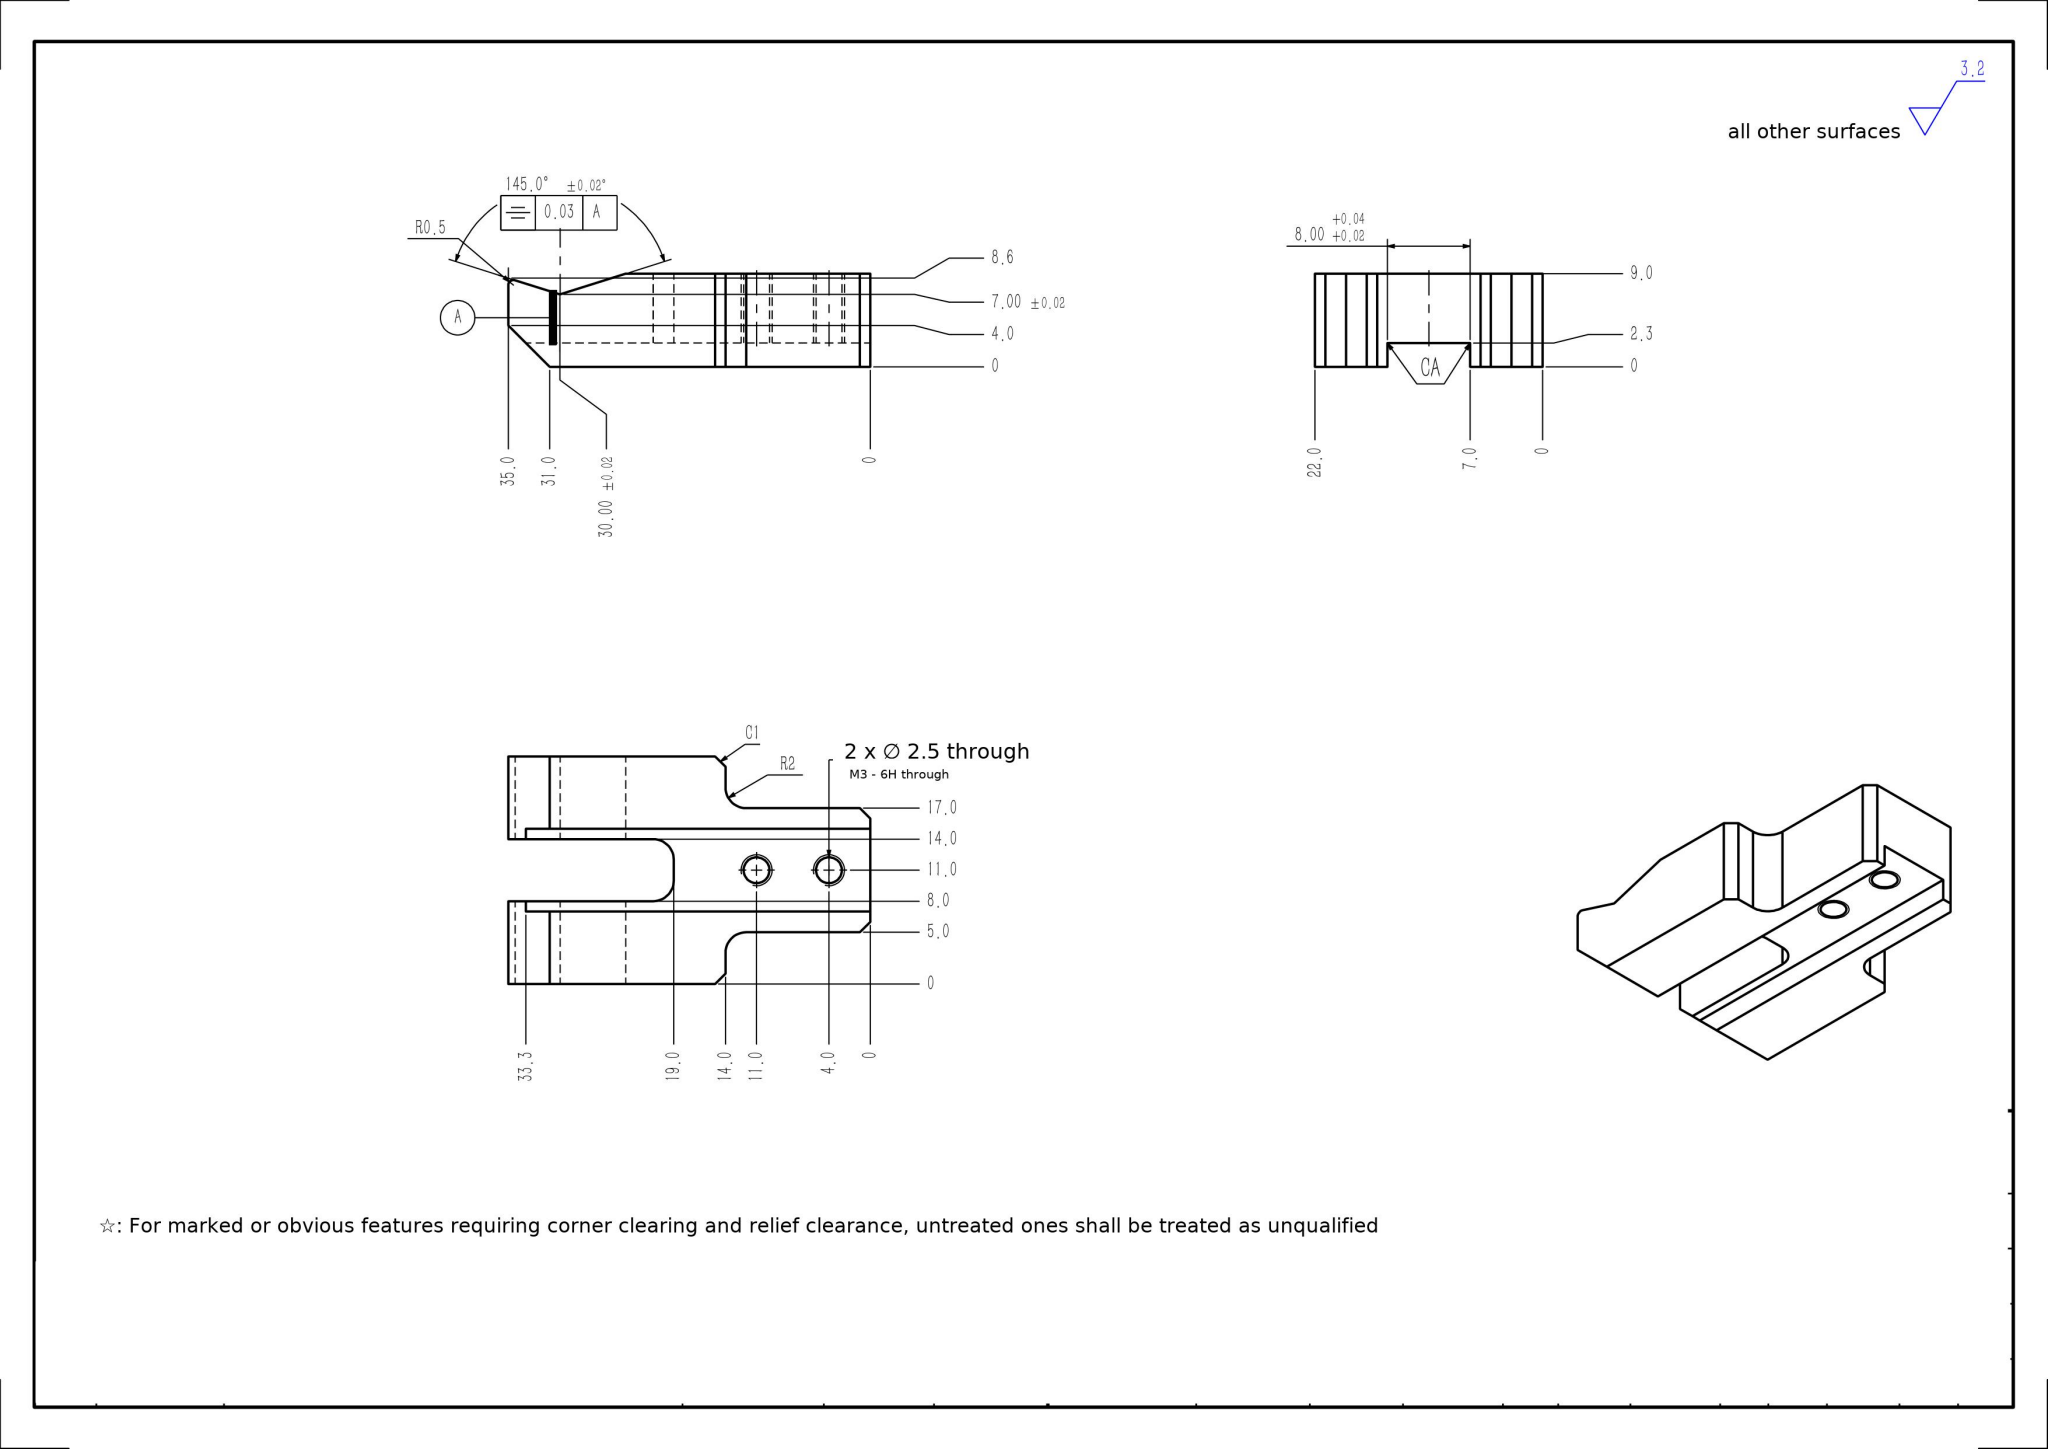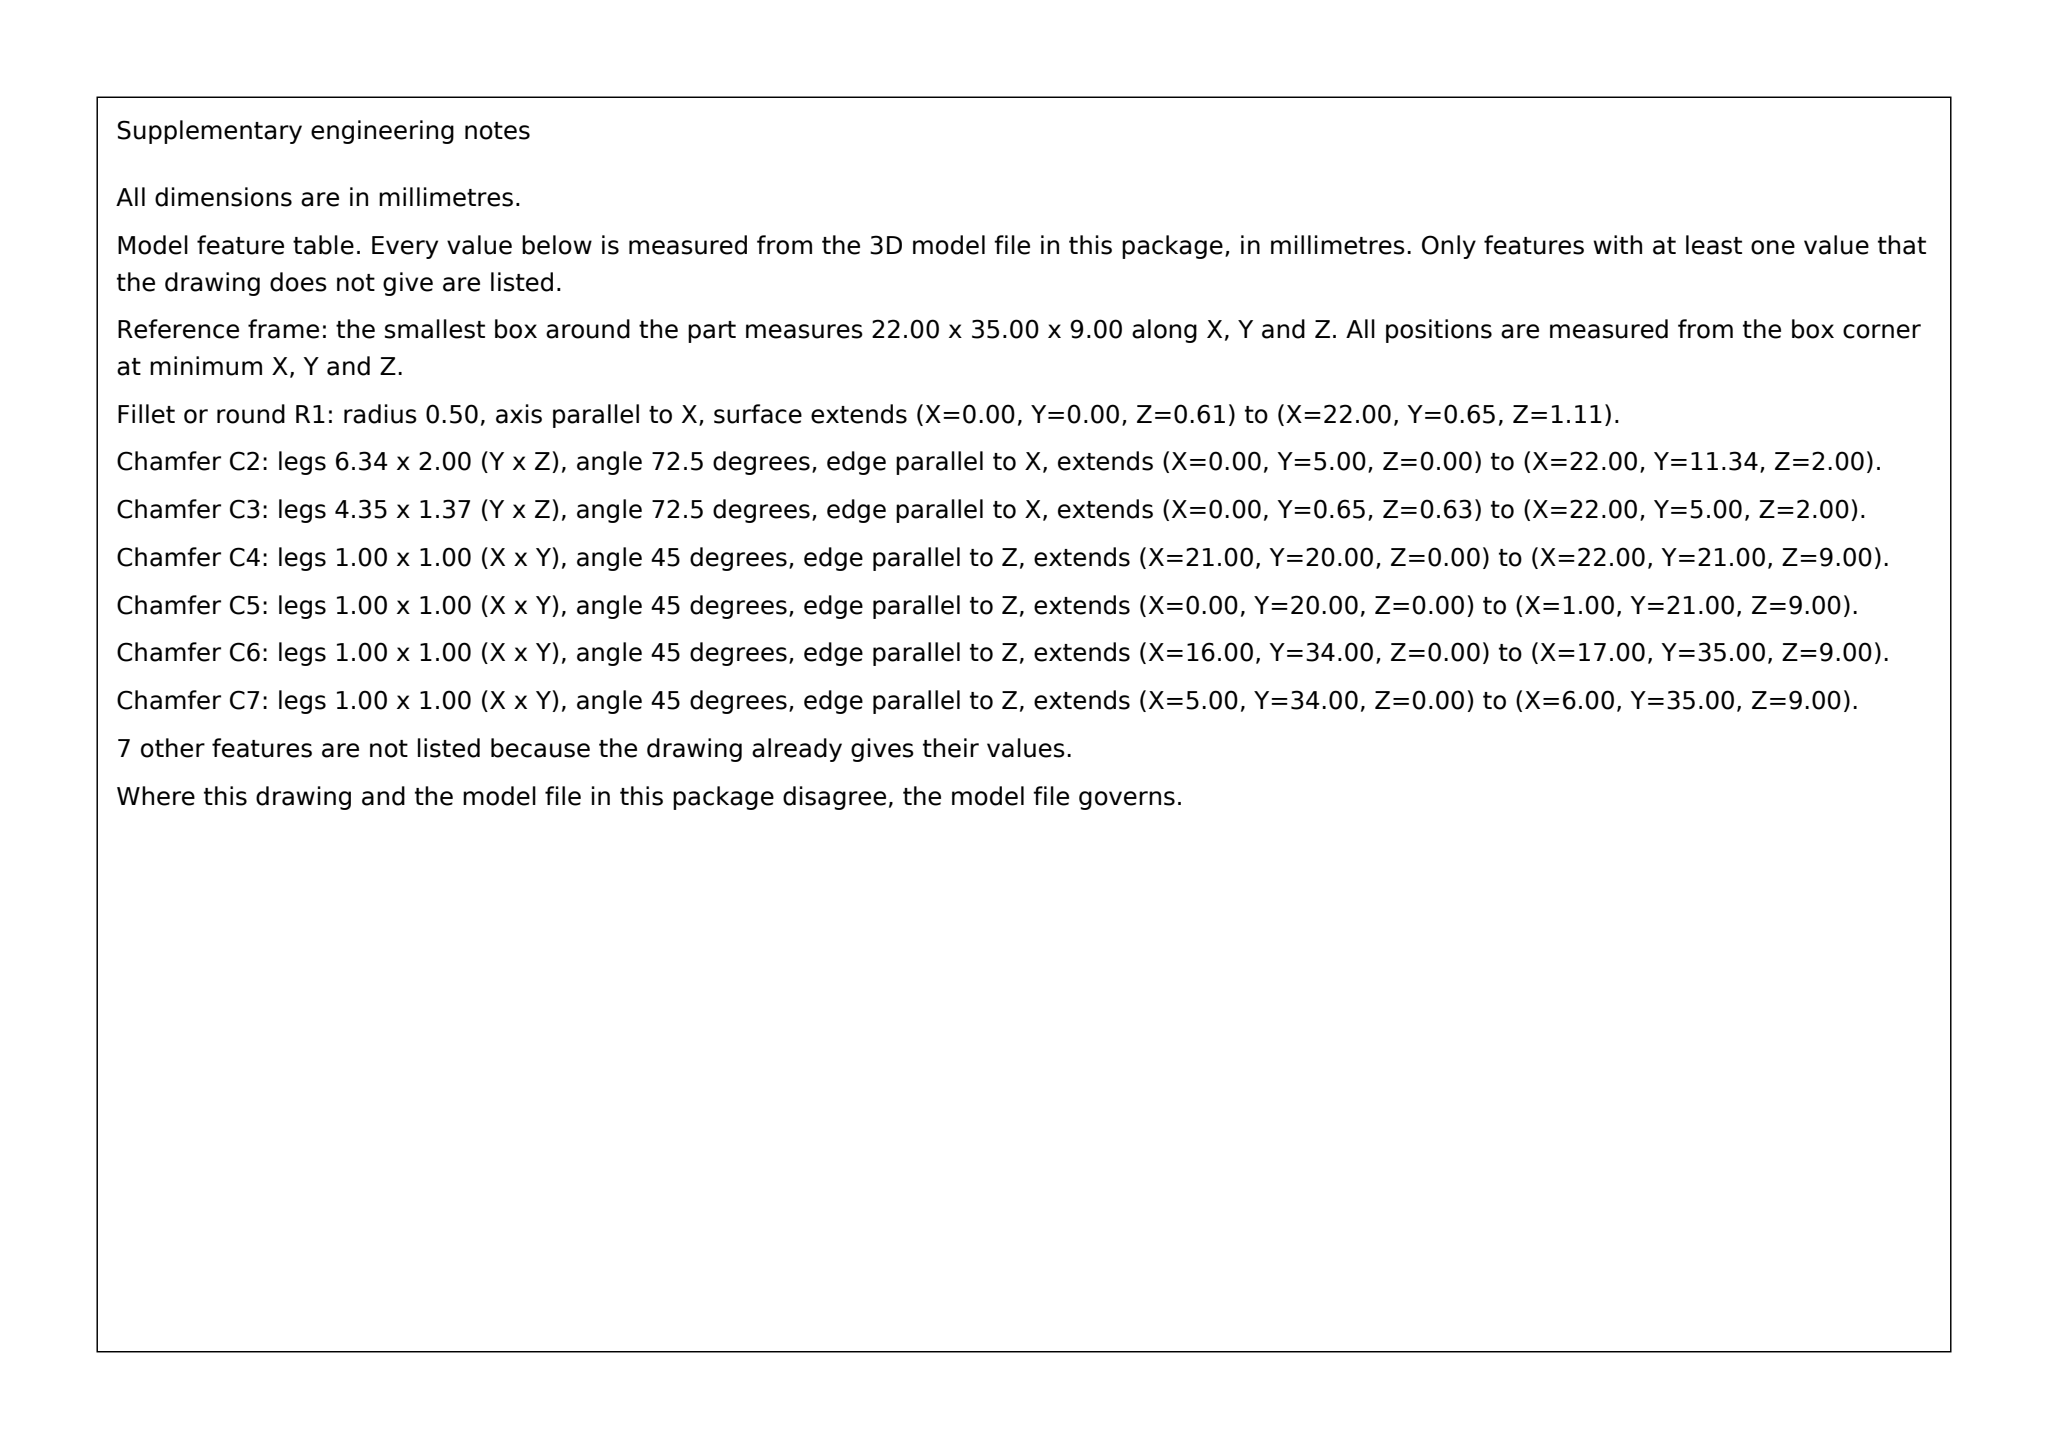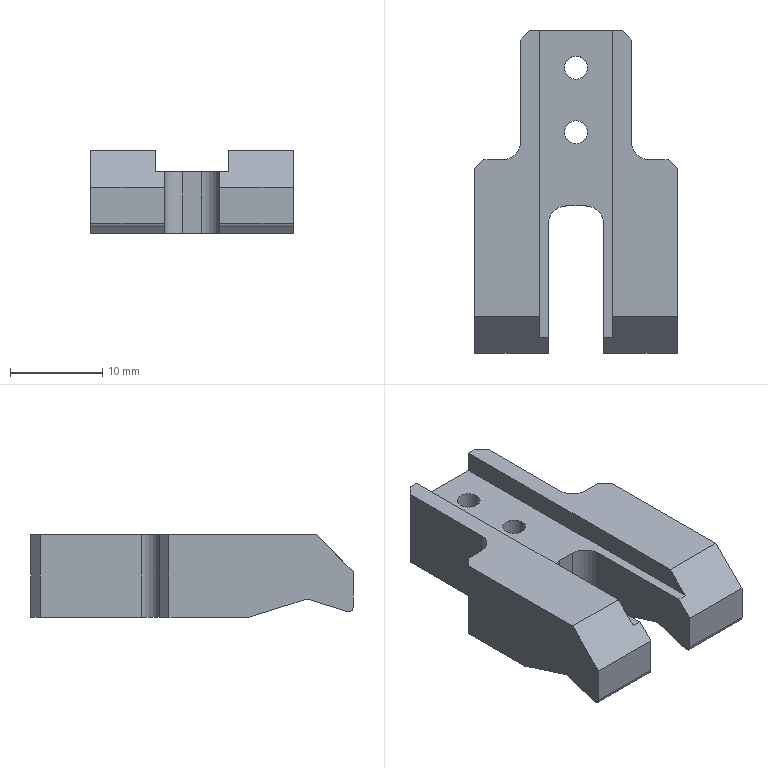Part | SolidWorks | mm | 1 solid | 40 faces | box 22 x 35 x 9 mm | volume 4011 mm3 | plane 28 | cylinder 12 | commonest cylinder face diameters 1 x4 2.5 x4 4 x4
build123d program:
from build123d import *

# Parameters (mm, degrees)
SKETCH1_W           = 22
SKETCH1_H           = 35
BOSS_EXTRUDE1_DEPTH = 9
SKETCH2_W           = 6
SKETCH2_H           = 16
CUT_EXTRUDE1_DEPTH  = 43.308
CUT_EXTRUDE2_DEPTH  = 43.308
SKETCH4_W           = 8
SKETCH4_H           = 42.52
CUT_EXTRUDE3_DEPTH  = 2.3
M3_TAPPED_HOLE1_D   = 2.5
SKETCH7_W           = 5
SKETCH7_H           = 14
CUT_EXTRUDE4_DEPTH  = 43.308
FILLET1_SIZE        = 1
CHAMFER1_SIZE       = 1
CHAMFER2_SIZE       = 4
FILLET2_R           = 2
FILLET3_R           = 2
FILLET4_R           = 0.5


with BuildPart() as part:
    # Sketch1 → Boss-Extrude1 (new body)
    with BuildSketch(Plane.XY):
        with Locations((11, -17.5)):
            Rectangle(SKETCH1_W, SKETCH1_H)
    extrude(amount=BOSS_EXTRUDE1_DEPTH)

    # Sketch2 → Cut-Extrude1 (cut, through all)
    with BuildSketch(Plane.XY.offset(9)):
        with Locations((11, -27)):
            Rectangle(SKETCH2_W, SKETCH2_H)
    extrude(amount=-CUT_EXTRUDE1_DEPTH, mode=Mode.SUBTRACT)

    # Sketch3 → Cut-Extrude2 (cut, through all)
    with BuildSketch(Plane(origin=(22, 0, 0), x_dir=(0, 0, -1), z_dir=(1, 0, 0))):
        Polygon((0, -23.657), (-2, -30), (0, -36.343), align=None)
    extrude(amount=-CUT_EXTRUDE2_DEPTH, mode=Mode.SUBTRACT)

    # Sketch4 → Cut-Extrude3 (cut)
    with BuildSketch(Plane.XY.offset(9)):
        with Locations((11, -21.26)):
            Rectangle(SKETCH4_W, SKETCH4_H)
    extrude(amount=-CUT_EXTRUDE3_DEPTH, mode=Mode.SUBTRACT)

    # M3 Tapped Hole1 (through all)
    with Locations(Plane.XY.offset(6.7)):
        with Locations((11, -4), (11, -11)):
            Hole(M3_TAPPED_HOLE1_D / 2)

    # Sketch7 → Cut-Extrude4 (cut, through all)
    with BuildSketch(Plane.XY.offset(9)):
        with Locations((19.5, -7)):
            Rectangle(SKETCH7_W, SKETCH7_H)
        with Locations((2.5, -7)):
            Rectangle(SKETCH7_W, SKETCH7_H)
    extrude(amount=-CUT_EXTRUDE4_DEPTH, mode=Mode.SUBTRACT)

    # Fillet1
    fillet1_edges = [part.edges().sort_by_distance(p)[0] for p in [
        (22, -14, 4.5),
        (0, -14, 4.5),
    ]]
    chamfer(fillet1_edges, length=FILLET1_SIZE)

    # Chamfer1
    chamfer1_edges = [part.edges().sort_by_distance(p)[0] for p in [
        (17, 0, 4.5),
        (5, 0, 4.5),
    ]]
    chamfer(chamfer1_edges, length=CHAMFER1_SIZE)

    # Chamfer2
    chamfer2_edges = [part.edges().sort_by_distance(p)[0] for p in [
        (3.5, -35, 9),
        (18.5, -35, 9),
    ]]
    chamfer(chamfer2_edges, length=CHAMFER2_SIZE)

    # Fillet2
    fillet2_edges = [part.edges().sort_by_distance(p)[0] for p in [
        (8, -19, 3.35),
        (14, -19, 3.35),
    ]]
    fillet(fillet2_edges, radius=FILLET2_R)

    # Fillet3
    fillet3_edges = [part.edges().sort_by_distance(p)[0] for p in [
        (17, -14, 4.5),
        (5, -14, 4.5),
    ]]
    fillet(fillet3_edges, radius=FILLET3_R)

    # Fillet4
    fillet4_edges = [part.edges().sort_by_distance(p)[0] for p in [
        (4, -35, 0.4235),
        (18, -35, 0.4235),
    ]]
    fillet(fillet4_edges, radius=FILLET4_R)


solid = part.part